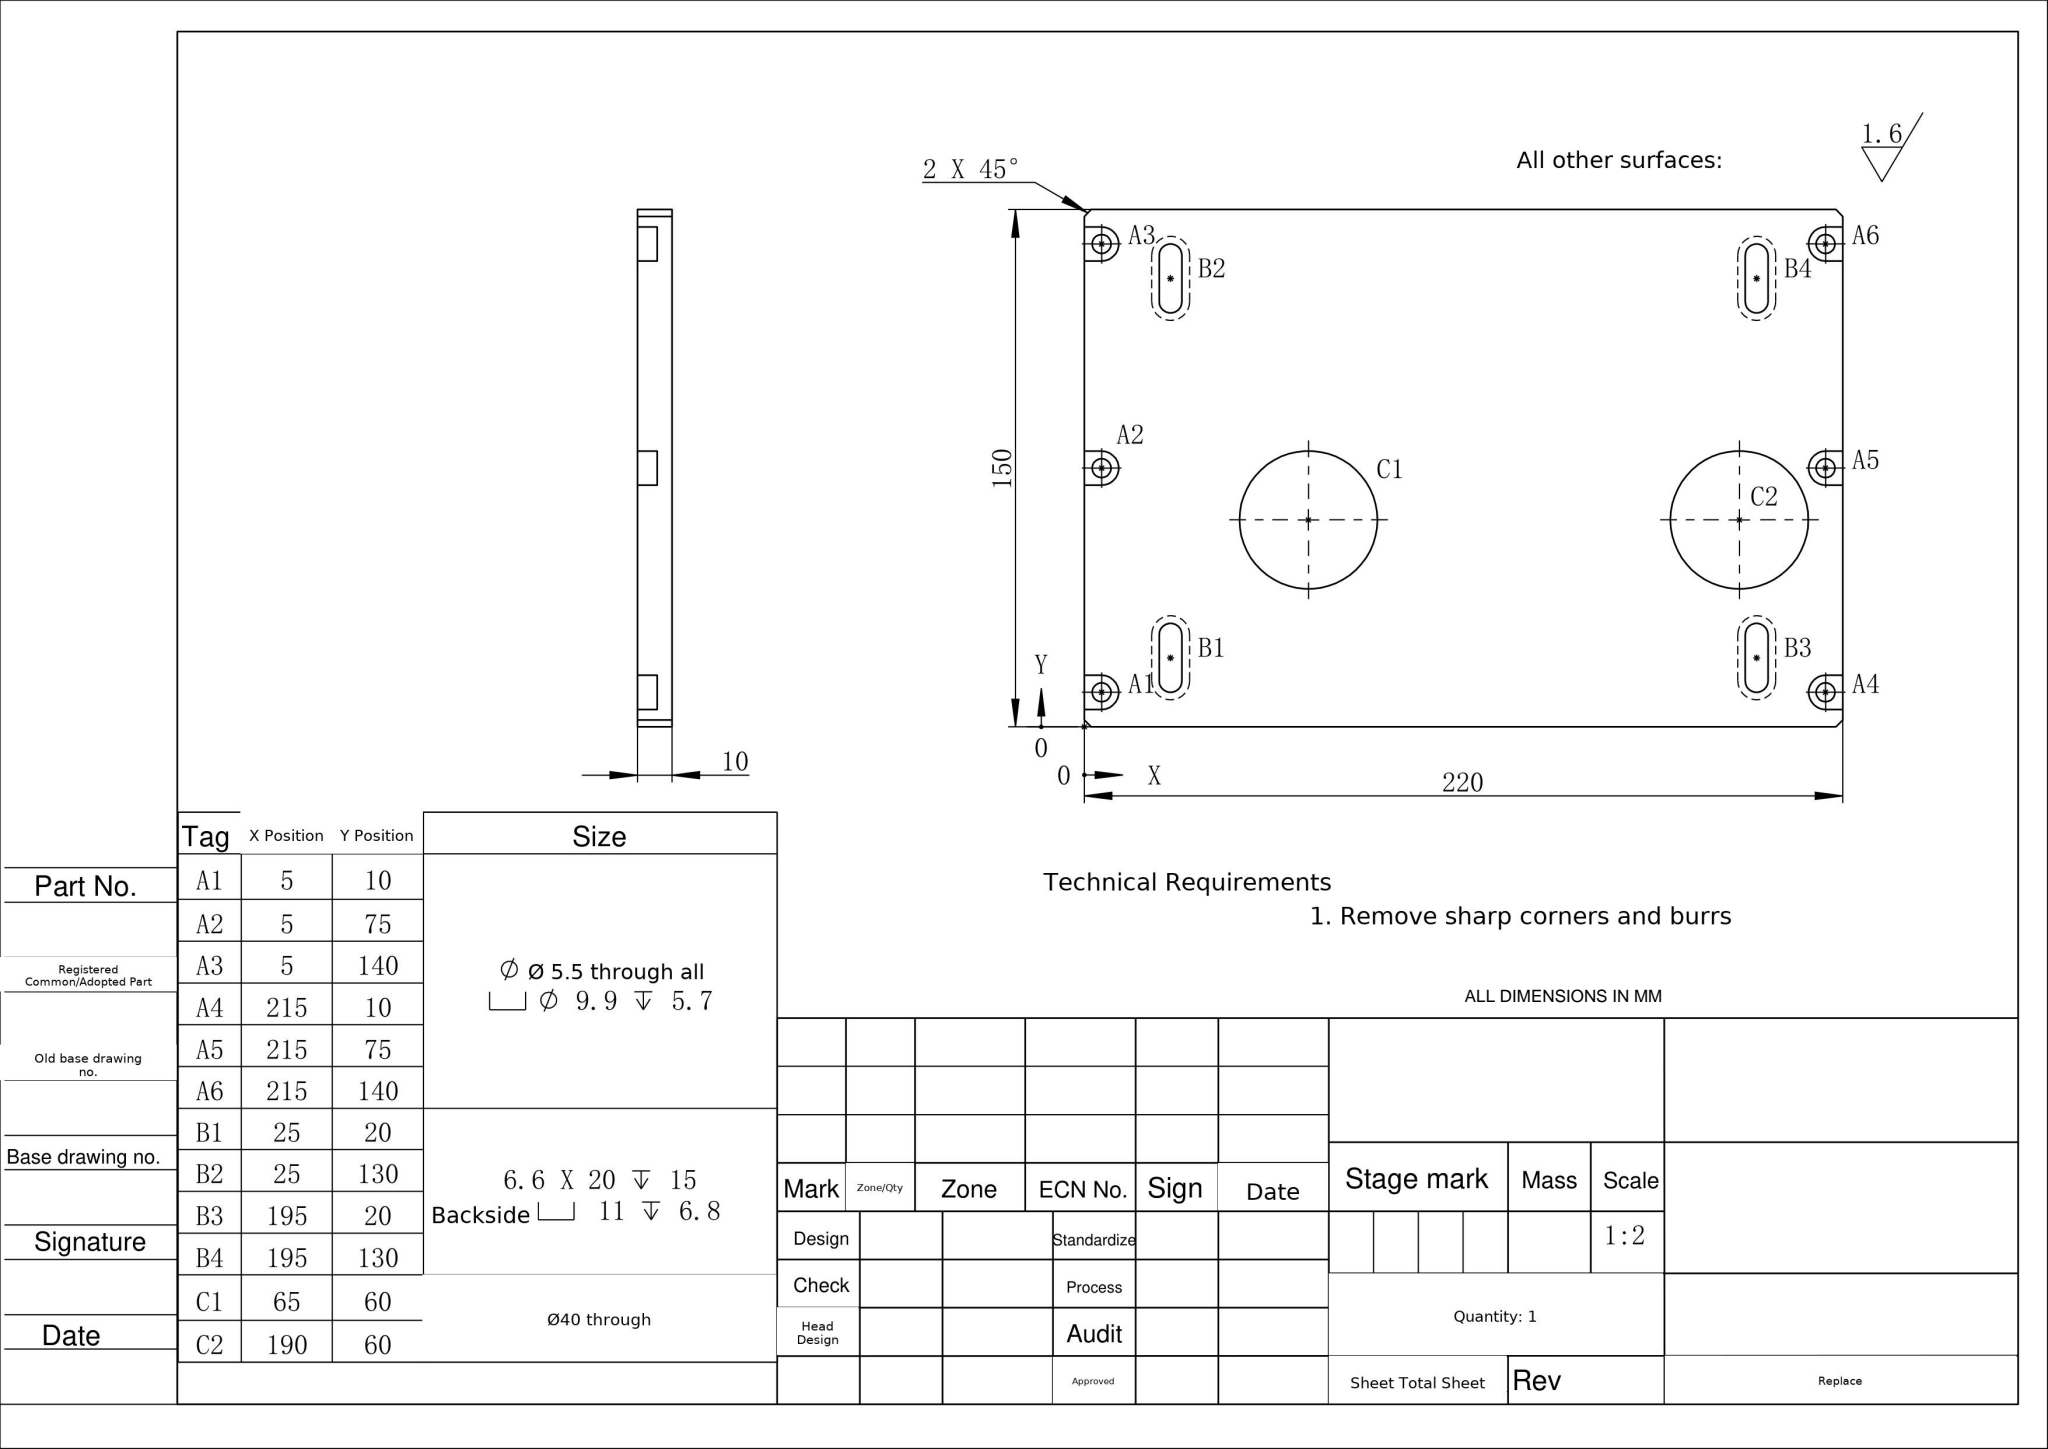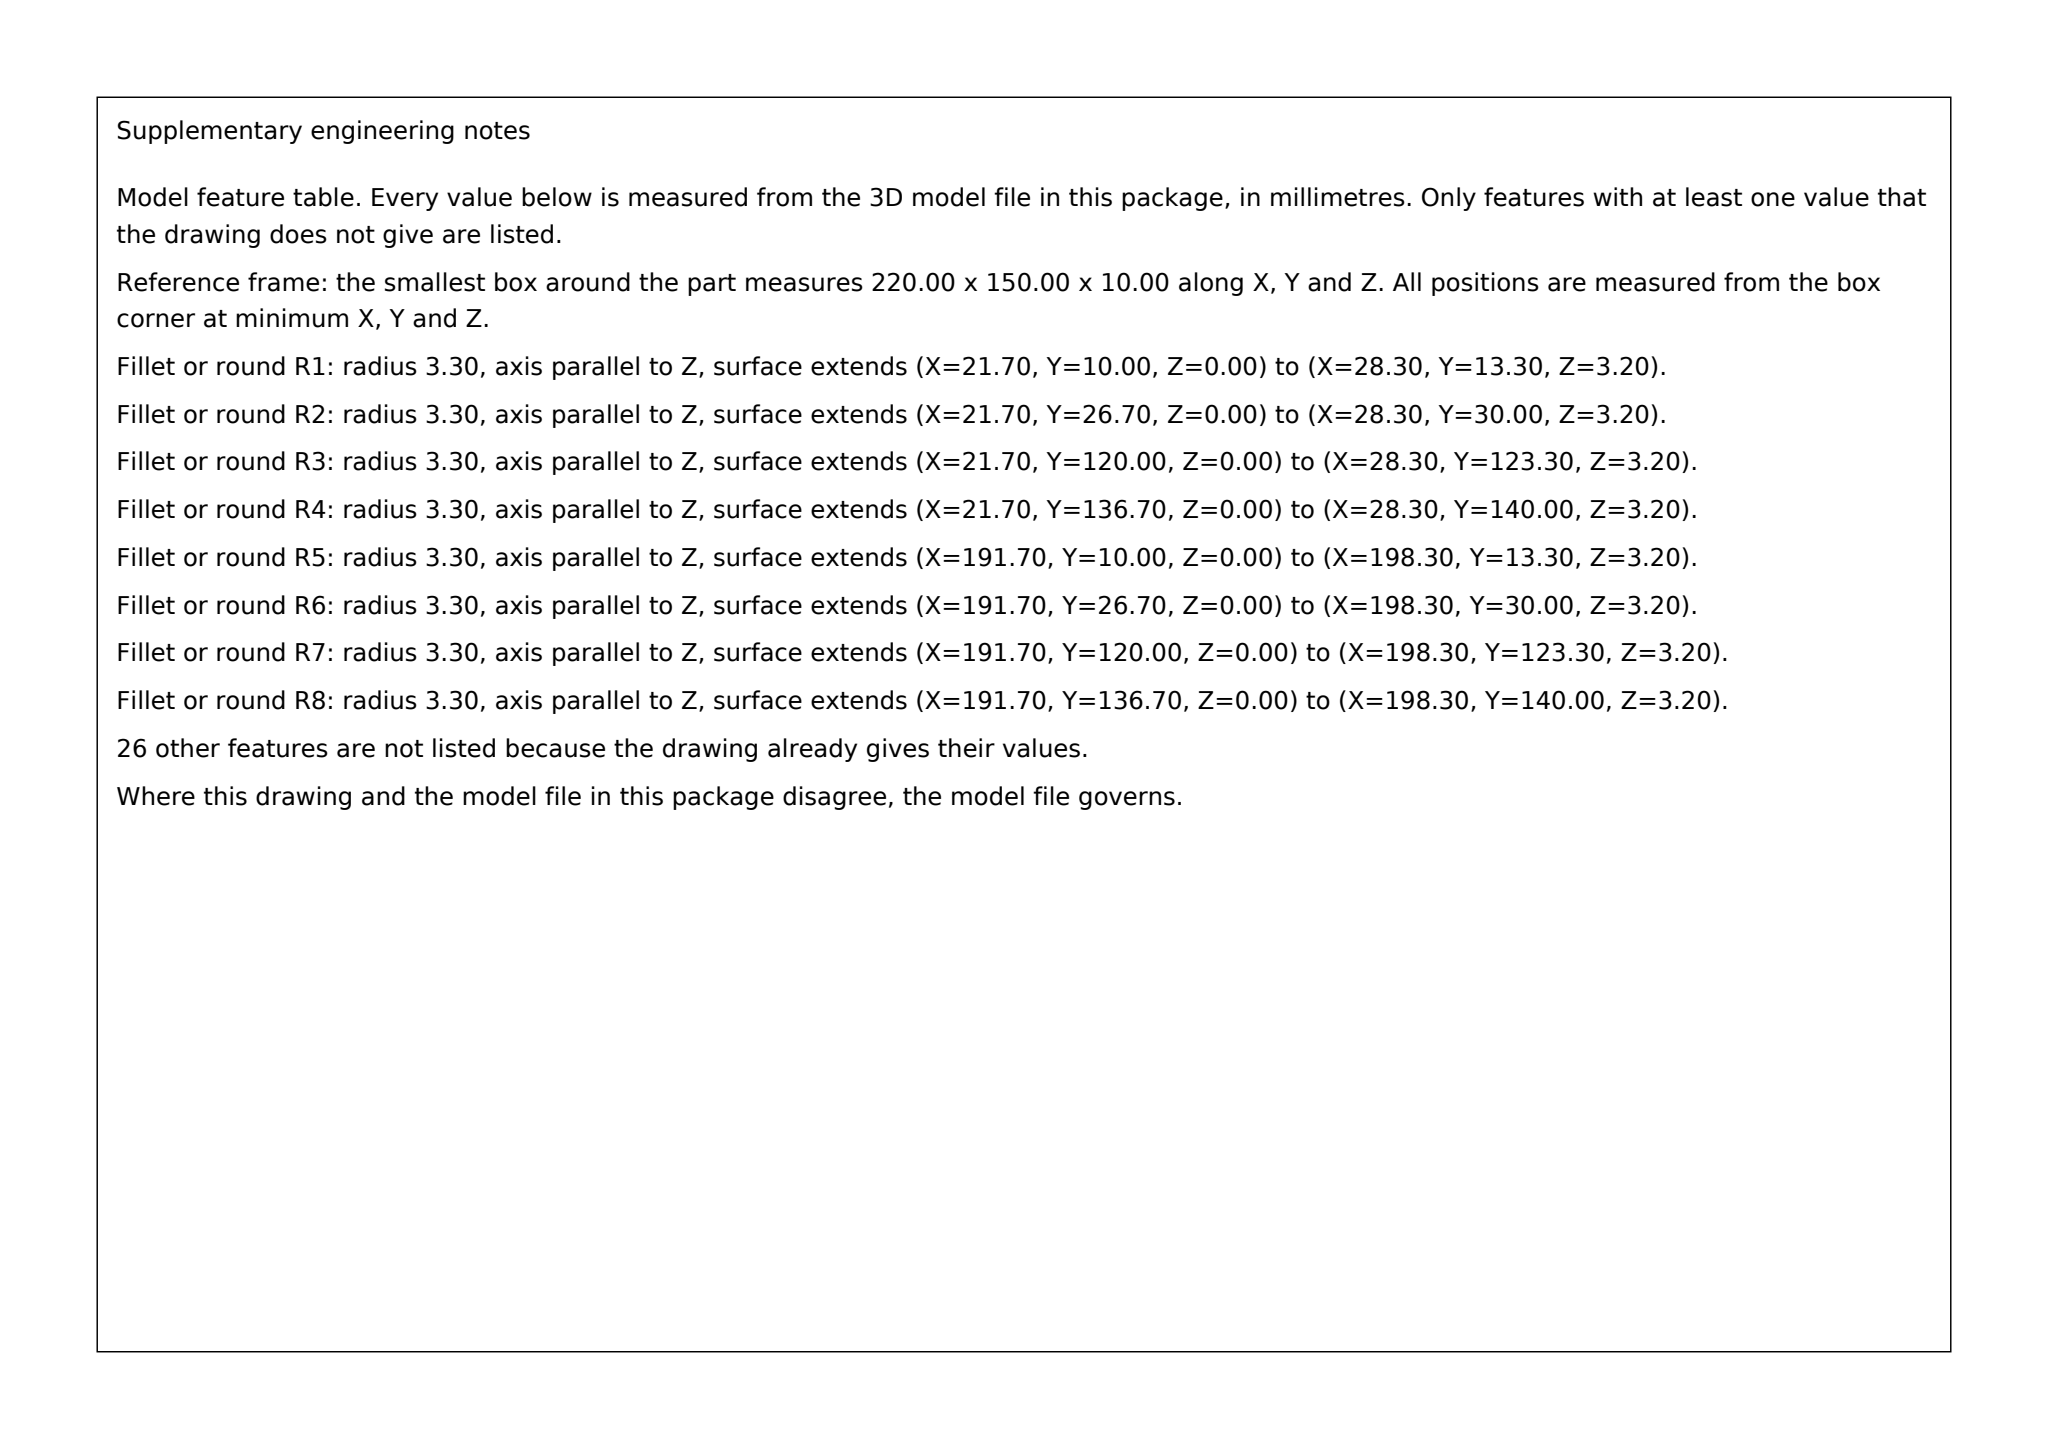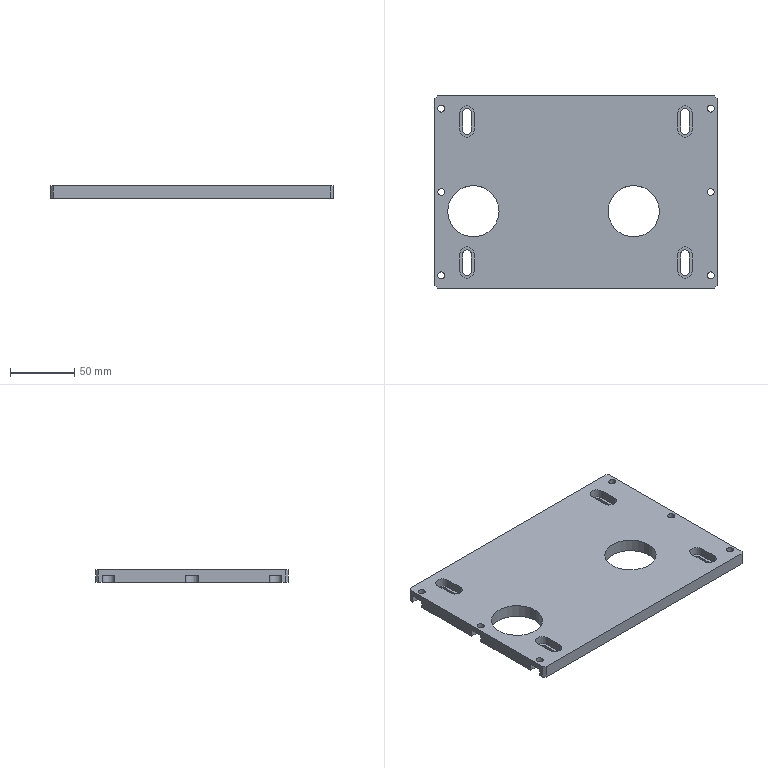Part | SolidWorks | mm | 1 solid | 89 faces | box 220 x 150 x 10 mm | volume 293001 mm3 | plane 48 | cylinder 41 | commonest cylinder face diameters 5.5 x12 9.9 x9 6.6 x8 11 x8 40 x4